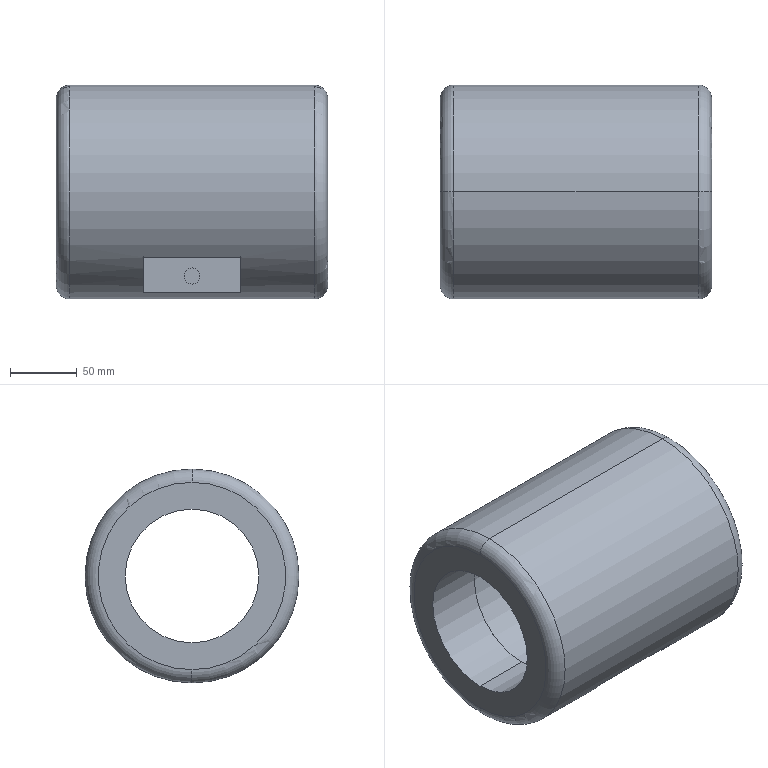Component | SolidWorks | CamMachineCasing-1 | 1 solid | 28 faces | box 203 x 160 x 160 mm | volume 2105138 mm3 | cylinder 10 | plane 10 | torus 8 | commonest cylinder face diameters 100 x4 12 x2 160 x2 112 x2
build123d program:
from build123d import *

# Parameters (mm, degrees)
SKETCH5_W          = 35
SKETCH5_H          = 72.809
CUT_EXTRUDE5_DEPTH = 120
SKETCH6_R          = 6
CUT_EXTRUDE6_DEPTH = 20


with BuildPart() as part:
    # Sketch1 → Revolve1 (revolve)
    with BuildSketch(Plane(origin=(0, 0, 0), x_dir=(0, 0, -1), z_dir=(1, 0, 0))):
        with BuildLine():
            Line((-56, -48), (-56, -155))
            ThreePointArc((-56, -155), (-54.828, -157.828), (-52, -159))
            Line((-52, -159), (-50, -159))
            Line((-50, -159), (-50, -203))
            Line((-50, -203), (-70, -203))
            ThreePointArc((-70, -203), (-77.071, -200.071), (-80, -193))
            Line((-80, -193), (-80, -10))
            ThreePointArc((-80, -10), (-77.071, -2.929), (-70, 0))
            Line((-70, 0), (-50, 0))
            Line((-50, 0), (-50, -44))
            Line((-50, -44), (-52, -44))
            ThreePointArc((-52, -44), (-54.828, -45.172), (-56, -48))
        make_face()
    revolve(axis=Axis((0, 0, 0), (0, -1, 0)))

    # Sketch5 → Cut-Extrude5 (cut)
    with BuildSketch(Plane(origin=(0, 0, -80), x_dir=(-1, 0, 0), z_dir=(0, 0, -1))):
        with Locations((45.79, -101.5)):
            Rectangle(SKETCH5_W, SKETCH5_H)
    extrude(amount=-CUT_EXTRUDE5_DEPTH, mode=Mode.SUBTRACT)

    # Sketch6 → Cut-Extrude6 (cut)
    with BuildSketch(Plane.ZY.offset(28.29)):
        with Locations((-62.831, -101.5)):
            Circle(SKETCH6_R)
    extrude(amount=-CUT_EXTRUDE6_DEPTH, mode=Mode.SUBTRACT)


solid = part.part

# Placed as in the assembly
solid = solid.moved(Location((587.733, 15.31, -110), (0, 0, 90)))
STEP:
#1=COLOUR_RGB('',0.7922,0.8196,0.9333);
#2=FILL_AREA_STYLE_COLOUR('',#1);
#3=FILL_AREA_STYLE('',(#2));
#4=SURFACE_STYLE_FILL_AREA(#3);
#5=SURFACE_SIDE_STYLE('',(#4));
#6=SURFACE_STYLE_USAGE(.BOTH.,#5);
#7=PRESENTATION_STYLE_ASSIGNMENT((#6));
#8=CARTESIAN_POINT('',(27.135,0.2764,-7.041));
#9=VERTEX_POINT('',#8);
#10=CARTESIAN_POINT('',(27.135,0.2764,-6.568));
#11=VERTEX_POINT('',#10);
#12=CARTESIAN_POINT('',(27.135,0.2764,-6.804));
#13=DIRECTION('',(0.,-1.,-0.));
#14=DIRECTION('',(0.,-0.,1.));
#15=AXIS2_PLACEMENT_3D('',#12,#13,#14);
#16=CIRCLE('',#15,0.2362);
#17=EDGE_CURVE('',#9,#11,#16,.T.);
#18=ORIENTED_EDGE('',*,*,#17,.F.);
#19=CARTESIAN_POINT('',(27.135,-0.511,-7.041));
#20=VERTEX_POINT('',#19);
#21=CARTESIAN_POINT('',(27.135,0.2764,-7.041));
#22=DIRECTION('',(0.,-1.,-0.));
#23=VECTOR('',#22,39.37);
#24=LINE('',#21,#23);
#25=EDGE_CURVE('',#9,#20,#24,.T.);
#26=ORIENTED_EDGE('',*,*,#25,.T.);
#27=CARTESIAN_POINT('',(27.135,-0.511,-6.568));
#28=VERTEX_POINT('',#27);
#29=CARTESIAN_POINT('',(27.135,-0.511,-6.804));
#30=DIRECTION('',(0.,-1.,-0.));
#31=DIRECTION('',(0.,0.,1.));
#32=AXIS2_PLACEMENT_3D('',#29,#30,#31);
#33=CIRCLE('',#32,0.2362);
#34=EDGE_CURVE('',#20,#28,#33,.T.);
#35=ORIENTED_EDGE('',*,*,#34,.T.);
#36=CARTESIAN_POINT('',(27.135,0.2764,-6.568));
#37=DIRECTION('',(0.,-1.,-0.));
#38=VECTOR('',#37,39.37);
#39=LINE('',#36,#38);
#40=EDGE_CURVE('',#11,#28,#39,.T.);
#41=ORIENTED_EDGE('',*,*,#40,.F.);
#42=EDGE_LOOP('',(#18,#26,#35,#41));
#43=FACE_OUTER_BOUND('',#42,.T.);
#44=CARTESIAN_POINT('',(27.135,0.2764,-6.804));
#45=DIRECTION('',(0.,-1.,-0.));
#46=DIRECTION('',(0.,-0.,1.));
#47=AXIS2_PLACEMENT_3D('',#44,#45,#46);
#48=CYLINDRICAL_SURFACE('',#47,0.2362);
#49=ADVANCED_FACE('',(#43),#48,.F.);
#50=CARTESIAN_POINT('',(29.399,0.6028,-6.378));
#51=VERTEX_POINT('',#50);
#52=CARTESIAN_POINT('',(29.399,0.6028,-2.283));
#53=VERTEX_POINT('',#52);
#54=CARTESIAN_POINT('',(29.399,0.6028,-4.331));
#55=DIRECTION('',(-1.,0.,0.));
#56=DIRECTION('',(0.,-0.,1.));
#57=AXIS2_PLACEMENT_3D('',#54,#55,#56);
#58=CIRCLE('',#57,2.047);
#59=EDGE_CURVE('',#51,#53,#58,.T.);
#60=ORIENTED_EDGE('',*,*,#59,.F.);
#61=CARTESIAN_POINT('',(29.241,0.6028,-6.535));
#62=VERTEX_POINT('',#61);
#63=CARTESIAN_POINT('',(29.241,0.6028,-6.378));
#64=DIRECTION('',(0.,1.,0.));
#65=DIRECTION('',(0.,-0.,1.));
#66=AXIS2_PLACEMENT_3D('',#63,#64,#65);
#67=CIRCLE('',#66,0.1575);
#68=EDGE_CURVE('',#51,#62,#67,.T.);
#69=ORIENTED_EDGE('',*,*,#68,.T.);
#70=CARTESIAN_POINT('',(29.241,0.6028,-2.126));
#71=VERTEX_POINT('',#70);
#72=CARTESIAN_POINT('',(29.241,0.6028,-4.331));
#73=DIRECTION('',(-1.,0.,0.));
#74=DIRECTION('',(0.,-0.,1.));
#75=AXIS2_PLACEMENT_3D('',#72,#73,#74);
#76=CIRCLE('',#75,2.205);
#77=EDGE_CURVE('',#62,#71,#76,.T.);
#78=ORIENTED_EDGE('',*,*,#77,.T.);
#79=CARTESIAN_POINT('',(29.241,0.6028,-2.283));
#80=DIRECTION('',(0.,-1.,-0.));
#81=DIRECTION('',(0.,0.,-1.));
#82=AXIS2_PLACEMENT_3D('',#79,#80,#81);
#83=CIRCLE('',#82,0.1575);
#84=EDGE_CURVE('',#53,#71,#83,.T.);
#85=ORIENTED_EDGE('',*,*,#84,.F.);
#86=EDGE_LOOP('',(#60,#69,#78,#85));
#87=FACE_OUTER_BOUND('',#86,.T.);
#88=CARTESIAN_POINT('',(29.241,0.6028,-4.331));
#89=DIRECTION('',(-1.,0.,0.));
#90=DIRECTION('',(0.,-0.,1.));
#91=AXIS2_PLACEMENT_3D('',#88,#89,#90);
#92=TOROIDAL_SURFACE('',#91,2.047,0.1575);
#93=ADVANCED_FACE('',(#87),#92,.F.);
#94=CARTESIAN_POINT('',(31.131,0.6028,-6.299));
#95=VERTEX_POINT('',#94);
#96=CARTESIAN_POINT('',(31.131,0.6028,-2.362));
#97=VERTEX_POINT('',#96);
#98=CARTESIAN_POINT('',(31.131,0.6028,-4.331));
#99=DIRECTION('',(-1.,0.,0.));
#100=DIRECTION('',(0.,-0.,1.));
#101=AXIS2_PLACEMENT_3D('',#98,#99,#100);
#102=CIRCLE('',#101,1.969);
#103=EDGE_CURVE('',#95,#97,#102,.T.);
#104=ORIENTED_EDGE('',*,*,#103,.F.);
#105=CARTESIAN_POINT('',(29.399,0.6028,-6.299));
#106=VERTEX_POINT('',#105);
#107=CARTESIAN_POINT('',(23.139,0.6028,-6.299));
#108=DIRECTION('',(-1.,0.,0.));
#109=VECTOR('',#108,39.37);
#110=LINE('',#107,#109);
#111=EDGE_CURVE('',#95,#106,#110,.T.);
#112=ORIENTED_EDGE('',*,*,#111,.T.);
#113=CARTESIAN_POINT('',(29.399,0.6028,-2.362));
#114=VERTEX_POINT('',#113);
#115=CARTESIAN_POINT('',(29.399,0.6028,-4.331));
#116=DIRECTION('',(-1.,0.,0.));
#117=DIRECTION('',(0.,-0.,1.));
#118=AXIS2_PLACEMENT_3D('',#115,#116,#117);
#119=CIRCLE('',#118,1.969);
#120=EDGE_CURVE('',#106,#114,#119,.T.);
#121=ORIENTED_EDGE('',*,*,#120,.T.);
#122=CARTESIAN_POINT('',(23.139,0.6028,-2.362));
#123=DIRECTION('',(-1.,0.,0.));
#124=VECTOR('',#123,39.37);
#125=LINE('',#122,#124);
#126=EDGE_CURVE('',#97,#114,#125,.T.);
#127=ORIENTED_EDGE('',*,*,#126,.F.);
#128=EDGE_LOOP('',(#104,#112,#121,#127));
#129=FACE_OUTER_BOUND('',#128,.T.);
#130=CARTESIAN_POINT('',(23.139,0.6028,-4.331));
#131=DIRECTION('',(-1.,0.,0.));
#132=DIRECTION('',(0.,-0.,1.));
#133=AXIS2_PLACEMENT_3D('',#130,#131,#132);
#134=CYLINDRICAL_SURFACE('',#133,1.969);
#135=ADVANCED_FACE('',(#129),#134,.F.);
#136=CARTESIAN_POINT('',(31.131,0.6028,-1.575));
#137=VERTEX_POINT('',#136);
#138=CARTESIAN_POINT('',(31.131,0.6028,-7.087));
#139=VERTEX_POINT('',#138);
#140=CARTESIAN_POINT('',(31.131,0.6028,-4.331));
#141=DIRECTION('',(-1.,0.,0.));
#142=DIRECTION('',(0.,-0.,1.));
#143=AXIS2_PLACEMENT_3D('',#140,#141,#142);
#144=CIRCLE('',#143,2.756);
#145=EDGE_CURVE('',#137,#139,#144,.T.);
#146=ORIENTED_EDGE('',*,*,#145,.T.);
#147=CARTESIAN_POINT('',(30.738,0.6028,-7.48));
#148=VERTEX_POINT('',#147);
#149=CARTESIAN_POINT('',(30.738,0.6028,-7.087));
#150=DIRECTION('',(0.,1.,0.));
#151=DIRECTION('',(0.,-0.,1.));
#152=AXIS2_PLACEMENT_3D('',#149,#150,#151);
#153=CIRCLE('',#152,0.3937);
#154=EDGE_CURVE('',#139,#148,#153,.T.);
#155=ORIENTED_EDGE('',*,*,#154,.T.);
#156=CARTESIAN_POINT('',(30.738,0.6028,-1.181));
#157=VERTEX_POINT('',#156);
#158=CARTESIAN_POINT('',(30.738,0.6028,-4.331));
#159=DIRECTION('',(-1.,0.,0.));
#160=DIRECTION('',(0.,-0.,1.));
#161=AXIS2_PLACEMENT_3D('',#158,#159,#160);
#162=CIRCLE('',#161,3.15);
#163=EDGE_CURVE('',#157,#148,#162,.T.);
#164=ORIENTED_EDGE('',*,*,#163,.F.);
#165=CARTESIAN_POINT('',(30.738,0.6028,-1.575));
#166=DIRECTION('',(0.,-1.,-0.));
#167=DIRECTION('',(0.,0.,-1.));
#168=AXIS2_PLACEMENT_3D('',#165,#166,#167);
#169=CIRCLE('',#168,0.3937);
#170=EDGE_CURVE('',#137,#157,#169,.T.);
#171=ORIENTED_EDGE('',*,*,#170,.F.);
#172=EDGE_LOOP('',(#146,#155,#164,#171));
#173=FACE_OUTER_BOUND('',#172,.T.);
#174=CARTESIAN_POINT('',(30.738,0.6028,-4.331));
#175=DIRECTION('',(-1.,0.,0.));
#176=DIRECTION('',(0.,-0.,1.));
#177=AXIS2_PLACEMENT_3D('',#174,#175,#176);
#178=TOROIDAL_SURFACE('',#177,2.756,0.3937);
#179=ADVANCED_FACE('',(#173),#178,.T.);
#180=ORIENTED_EDGE('',*,*,#163,.T.);
#181=CARTESIAN_POINT('',(23.533,0.6028,-7.48));
#182=VERTEX_POINT('',#181);
#183=CARTESIAN_POINT('',(23.139,0.6028,-7.48));
#184=DIRECTION('',(-1.,0.,0.));
#185=VECTOR('',#184,39.37);
#186=LINE('',#183,#185);
#187=EDGE_CURVE('',#148,#182,#186,.T.);
#188=ORIENTED_EDGE('',*,*,#187,.T.);
#189=CARTESIAN_POINT('',(23.533,0.6028,-1.181));
#190=VERTEX_POINT('',#189);
#191=CARTESIAN_POINT('',(23.533,0.6028,-4.331));
#192=DIRECTION('',(-1.,0.,0.));
#193=DIRECTION('',(0.,-0.,1.));
#194=AXIS2_PLACEMENT_3D('',#191,#192,#193);
#195=CIRCLE('',#194,3.15);
#196=EDGE_CURVE('',#190,#182,#195,.T.);
#197=ORIENTED_EDGE('',*,*,#196,.F.);
#198=CARTESIAN_POINT('',(23.139,0.6028,-1.181));
#199=DIRECTION('',(-1.,0.,0.));
#200=VECTOR('',#199,39.37);
#201=LINE('',#198,#200);
#202=EDGE_CURVE('',#157,#190,#201,.T.);
#203=ORIENTED_EDGE('',*,*,#202,.F.);
#204=EDGE_LOOP('',(#180,#188,#197,#203));
#205=FACE_OUTER_BOUND('',#204,.T.);
#206=CARTESIAN_POINT('',(23.139,0.6028,-4.331));
#207=DIRECTION('',(-1.,0.,0.));
#208=DIRECTION('',(0.,-0.,1.));
#209=AXIS2_PLACEMENT_3D('',#206,#207,#208);
#210=CYLINDRICAL_SURFACE('',#209,3.15);
#211=ADVANCED_FACE('',(#205),#210,.T.);
#212=ORIENTED_EDGE('',*,*,#196,.T.);
#213=CARTESIAN_POINT('',(23.139,0.6028,-7.087));
#214=VERTEX_POINT('',#213);
#215=CARTESIAN_POINT('',(23.533,0.6028,-7.087));
#216=DIRECTION('',(0.,1.,0.));
#217=DIRECTION('',(0.,-0.,1.));
#218=AXIS2_PLACEMENT_3D('',#215,#216,#217);
#219=CIRCLE('',#218,0.3937);
#220=EDGE_CURVE('',#182,#214,#219,.T.);
#221=ORIENTED_EDGE('',*,*,#220,.T.);
#222=CARTESIAN_POINT('',(23.139,0.6028,-1.575));
#223=VERTEX_POINT('',#222);
#224=CARTESIAN_POINT('',(23.139,0.6028,-4.331));
#225=DIRECTION('',(-1.,0.,0.));
#226=DIRECTION('',(0.,-0.,1.));
#227=AXIS2_PLACEMENT_3D('',#224,#225,#226);
#228=CIRCLE('',#227,2.756);
#229=EDGE_CURVE('',#223,#214,#228,.T.);
#230=ORIENTED_EDGE('',*,*,#229,.F.);
#231=CARTESIAN_POINT('',(23.533,0.6028,-1.575));
#232=DIRECTION('',(0.,-1.,-0.));
#233=DIRECTION('',(0.,0.,-1.));
#234=AXIS2_PLACEMENT_3D('',#231,#232,#233);
#235=CIRCLE('',#234,0.3937);
#236=EDGE_CURVE('',#190,#223,#235,.T.);
#237=ORIENTED_EDGE('',*,*,#236,.F.);
#238=EDGE_LOOP('',(#212,#221,#230,#237));
#239=FACE_OUTER_BOUND('',#238,.T.);
#240=CARTESIAN_POINT('',(23.533,0.6028,-4.331));
#241=DIRECTION('',(-1.,0.,0.));
#242=DIRECTION('',(0.,-0.,1.));
#243=AXIS2_PLACEMENT_3D('',#240,#241,#242);
#244=TOROIDAL_SURFACE('',#243,2.756,0.3937);
#245=ADVANCED_FACE('',(#239),#244,.T.);
#246=CARTESIAN_POINT('',(24.871,0.6028,-6.299));
#247=VERTEX_POINT('',#246);
#248=CARTESIAN_POINT('',(24.871,0.6028,-2.362));
#249=VERTEX_POINT('',#248);
#250=CARTESIAN_POINT('',(24.871,0.6028,-4.331));
#251=DIRECTION('',(-1.,0.,0.));
#252=DIRECTION('',(0.,-0.,1.));
#253=AXIS2_PLACEMENT_3D('',#250,#251,#252);
#254=CIRCLE('',#253,1.969);
#255=EDGE_CURVE('',#247,#249,#254,.T.);
#256=ORIENTED_EDGE('',*,*,#255,.F.);
#257=CARTESIAN_POINT('',(23.139,0.6028,-6.299));
#258=VERTEX_POINT('',#257);
#259=CARTESIAN_POINT('',(23.139,0.6028,-6.299));
#260=DIRECTION('',(-1.,0.,0.));
#261=VECTOR('',#260,39.37);
#262=LINE('',#259,#261);
#263=EDGE_CURVE('',#247,#258,#262,.T.);
#264=ORIENTED_EDGE('',*,*,#263,.T.);
#265=CARTESIAN_POINT('',(23.139,0.6028,-2.362));
#266=VERTEX_POINT('',#265);
#267=CARTESIAN_POINT('',(23.139,0.6028,-4.331));
#268=DIRECTION('',(-1.,0.,0.));
#269=DIRECTION('',(0.,-0.,1.));
#270=AXIS2_PLACEMENT_3D('',#267,#268,#269);
#271=CIRCLE('',#270,1.969);
#272=EDGE_CURVE('',#258,#266,#271,.T.);
#273=ORIENTED_EDGE('',*,*,#272,.T.);
#274=CARTESIAN_POINT('',(23.139,0.6028,-2.362));
#275=DIRECTION('',(-1.,0.,0.));
#276=VECTOR('',#275,39.37);
#277=LINE('',#274,#276);
#278=EDGE_CURVE('',#249,#266,#277,.T.);
#279=ORIENTED_EDGE('',*,*,#278,.F.);
#280=EDGE_LOOP('',(#256,#264,#273,#279));
#281=FACE_OUTER_BOUND('',#280,.T.);
#282=CARTESIAN_POINT('',(23.139,0.6028,-4.331));
#283=DIRECTION('',(-1.,0.,0.));
#284=DIRECTION('',(0.,-0.,1.));
#285=AXIS2_PLACEMENT_3D('',#282,#283,#284);
#286=CYLINDRICAL_SURFACE('',#285,1.969);
#287=ADVANCED_FACE('',(#281),#286,.F.);
#288=CARTESIAN_POINT('',(25.029,0.6028,-6.535));
#289=VERTEX_POINT('',#288);
#290=CARTESIAN_POINT('',(25.029,0.6028,-2.126));
#291=VERTEX_POINT('',#290);
#292=CARTESIAN_POINT('',(25.029,0.6028,-4.331));
#293=DIRECTION('',(-1.,0.,0.));
#294=DIRECTION('',(0.,-0.,1.));
#295=AXIS2_PLACEMENT_3D('',#292,#293,#294);
#296=CIRCLE('',#295,2.205);
#297=EDGE_CURVE('',#289,#291,#296,.T.);
#298=ORIENTED_EDGE('',*,*,#297,.F.);
#299=CARTESIAN_POINT('',(24.871,0.6028,-6.378));
#300=VERTEX_POINT('',#299);
#301=CARTESIAN_POINT('',(25.029,0.6028,-6.378));
#302=DIRECTION('',(0.,1.,0.));
#303=DIRECTION('',(0.,-0.,1.));
#304=AXIS2_PLACEMENT_3D('',#301,#302,#303);
#305=CIRCLE('',#304,0.1575);
#306=EDGE_CURVE('',#289,#300,#305,.T.);
#307=ORIENTED_EDGE('',*,*,#306,.T.);
#308=CARTESIAN_POINT('',(24.871,0.6028,-2.283));
#309=VERTEX_POINT('',#308);
#310=CARTESIAN_POINT('',(24.871,0.6028,-4.331));
#311=DIRECTION('',(-1.,0.,0.));
#312=DIRECTION('',(0.,-0.,1.));
#313=AXIS2_PLACEMENT_3D('',#310,#311,#312);
#314=CIRCLE('',#313,2.047);
#315=EDGE_CURVE('',#300,#309,#314,.T.);
#316=ORIENTED_EDGE('',*,*,#315,.T.);
#317=CARTESIAN_POINT('',(25.029,0.6028,-2.283));
#318=DIRECTION('',(0.,-1.,-0.));
#319=DIRECTION('',(0.,0.,-1.));
#320=AXIS2_PLACEMENT_3D('',#317,#318,#319);
#321=CIRCLE('',#320,0.1575);
#322=EDGE_CURVE('',#291,#309,#321,.T.);
#323=ORIENTED_EDGE('',*,*,#322,.F.);
#324=EDGE_LOOP('',(#298,#307,#316,#323));
#325=FACE_OUTER_BOUND('',#324,.T.);
#326=CARTESIAN_POINT('',(25.029,0.6028,-4.331));
#327=DIRECTION('',(-1.,0.,0.));
#328=DIRECTION('',(0.,-0.,1.));
#329=AXIS2_PLACEMENT_3D('',#326,#327,#328);
#330=TOROIDAL_SURFACE('',#329,2.047,0.1575);
#331=ADVANCED_FACE('',(#325),#330,.F.);
#332=CARTESIAN_POINT('',(25.702,-0.9402,-2.756));
#333=VERTEX_POINT('',#332);
#334=CARTESIAN_POINT('',(25.702,-0.511,-6.233));
#335=VERTEX_POINT('',#334);
#336=CARTESIAN_POINT('',(25.702,0.6028,-4.331));
#337=DIRECTION('',(1.,-0.,-0.));
#338=DIRECTION('',(0.,-1.,-0.));
#339=AXIS2_PLACEMENT_3D('',#336,#337,#338);
#340=CIRCLE('',#339,2.205);
#341=EDGE_CURVE('',#333,#335,#340,.T.);
#342=ORIENTED_EDGE('',*,*,#341,.T.);
#343=CARTESIAN_POINT('',(28.568,-0.511,-6.233));
#344=VERTEX_POINT('',#343);
#345=CARTESIAN_POINT('',(23.139,-0.511,-6.233));
#346=DIRECTION('',(1.,0.,0.));
#347=VECTOR('',#346,39.37);
#348=LINE('',#345,#347);
#349=EDGE_CURVE('',#335,#344,#348,.T.);
#350=ORIENTED_EDGE('',*,*,#349,.T.);
#351=CARTESIAN_POINT('',(28.568,-0.9402,-2.756));
#352=VERTEX_POINT('',#351);
#353=CARTESIAN_POINT('',(28.568,0.6028,-4.331));
#354=DIRECTION('',(-1.,0.,0.));
#355=DIRECTION('',(0.,0.,-1.));
#356=AXIS2_PLACEMENT_3D('',#353,#354,#355);
#357=CIRCLE('',#356,2.205);
#358=EDGE_CURVE('',#344,#352,#357,.T.);
#359=ORIENTED_EDGE('',*,*,#358,.T.);
#360=CARTESIAN_POINT('',(23.139,-0.9402,-2.756));
#361=DIRECTION('',(-1.,0.,0.));
#362=VECTOR('',#361,39.37);
#363=LINE('',#360,#362);
#364=EDGE_CURVE('',#352,#333,#363,.T.);
#365=ORIENTED_EDGE('',*,*,#364,.T.);
#366=EDGE_LOOP('',(#342,#350,#359,#365));
#367=FACE_BOUND('',#366,.T.);
#368=ORIENTED_EDGE('',*,*,#77,.F.);
#369=CARTESIAN_POINT('',(23.139,0.6028,-6.535));
#370=DIRECTION('',(-1.,0.,0.));
#371=VECTOR('',#370,39.37);
#372=LINE('',#369,#371);
#373=EDGE_CURVE('',#62,#289,#372,.T.);
#374=ORIENTED_EDGE('',*,*,#373,.T.);
#375=ORIENTED_EDGE('',*,*,#297,.T.);
#376=CARTESIAN_POINT('',(23.139,0.6028,-2.126));
#377=DIRECTION('',(-1.,0.,0.));
#378=VECTOR('',#377,39.37);
#379=LINE('',#376,#378);
#380=EDGE_CURVE('',#71,#291,#379,.T.);
#381=ORIENTED_EDGE('',*,*,#380,.F.);
#382=EDGE_LOOP('',(#368,#374,#375,#381));
#383=FACE_OUTER_BOUND('',#382,.T.);
#384=CARTESIAN_POINT('',(23.139,0.6028,-4.331));
#385=DIRECTION('',(-1.,0.,0.));
#386=DIRECTION('',(0.,-0.,1.));
#387=AXIS2_PLACEMENT_3D('',#384,#385,#386);
#388=CYLINDRICAL_SURFACE('',#387,2.205);
#389=ADVANCED_FACE('',(#367,#383),#388,.F.);
#390=ORIENTED_EDGE('',*,*,#373,.F.);
#391=CARTESIAN_POINT('',(29.241,0.6028,-4.331));
#392=DIRECTION('',(-1.,0.,0.));
#393=DIRECTION('',(0.,-0.,1.));
#394=AXIS2_PLACEMENT_3D('',#391,#392,#393);
#395=CIRCLE('',#394,2.205);
#396=EDGE_CURVE('',#71,#62,#395,.T.);
#397=ORIENTED_EDGE('',*,*,#396,.F.);
#398=ORIENTED_EDGE('',*,*,#380,.T.);
#399=CARTESIAN_POINT('',(25.029,0.6028,-4.331));
#400=DIRECTION('',(-1.,0.,0.));
#401=DIRECTION('',(0.,-0.,1.));
#402=AXIS2_PLACEMENT_3D('',#399,#400,#401);
#403=CIRCLE('',#402,2.205);
#404=EDGE_CURVE('',#291,#289,#403,.T.);
#405=ORIENTED_EDGE('',*,*,#404,.T.);
#406=EDGE_LOOP('',(#390,#397,#398,#405));
#407=FACE_OUTER_BOUND('',#406,.T.);
#408=CARTESIAN_POINT('',(23.139,0.6028,-4.331));
#409=DIRECTION('',(-1.,0.,0.));
#410=DIRECTION('',(0.,-0.,1.));
#411=AXIS2_PLACEMENT_3D('',#408,#409,#410);
#412=CYLINDRICAL_SURFACE('',#411,2.205);
#413=ADVANCED_FACE('',(#407),#412,.F.);
#414=ORIENTED_EDGE('',*,*,#306,.F.);
#415=ORIENTED_EDGE('',*,*,#404,.F.);
#416=ORIENTED_EDGE('',*,*,#322,.T.);
#417=CARTESIAN_POINT('',(24.871,0.6028,-4.331));
#418=DIRECTION('',(-1.,0.,0.));
#419=DIRECTION('',(0.,-0.,1.));
#420=AXIS2_PLACEMENT_3D('',#417,#418,#419);
#421=CIRCLE('',#420,2.047);
#422=EDGE_CURVE('',#309,#300,#421,.T.);
#423=ORIENTED_EDGE('',*,*,#422,.T.);
#424=EDGE_LOOP('',(#414,#415,#416,#423));
#425=FACE_OUTER_BOUND('',#424,.T.);
#426=CARTESIAN_POINT('',(25.029,0.6028,-4.331));
#427=DIRECTION('',(-1.,0.,0.));
#428=DIRECTION('',(0.,-0.,1.));
#429=AXIS2_PLACEMENT_3D('',#426,#427,#428);
#430=TOROIDAL_SURFACE('',#429,2.047,0.1575);
#431=ADVANCED_FACE('',(#425),#430,.F.);
#432=ORIENTED_EDGE('',*,*,#422,.F.);
#433=ORIENTED_EDGE('',*,*,#315,.F.);
#434=EDGE_LOOP('',(#432,#433));
#435=FACE_OUTER_BOUND('',#434,.T.);
#436=CARTESIAN_POINT('',(24.871,0.6028,-4.331));
#437=DIRECTION('',(-1.,0.,0.));
#438=DIRECTION('',(0.,-0.,1.));
#439=AXIS2_PLACEMENT_3D('',#436,#437,#438);
#440=CIRCLE('',#439,1.969);
#441=EDGE_CURVE('',#249,#247,#440,.T.);
#442=ORIENTED_EDGE('',*,*,#441,.T.);
#443=ORIENTED_EDGE('',*,*,#255,.T.);
#444=EDGE_LOOP('',(#442,#443));
#445=FACE_BOUND('',#444,.T.);
#446=CARTESIAN_POINT('',(24.871,0.6028,-4.331));
#447=DIRECTION('',(-1.,0.,0.));
#448=DIRECTION('',(0.,-0.,1.));
#449=AXIS2_PLACEMENT_3D('',#446,#447,#448);
#450=PLANE('',#449);
#451=ADVANCED_FACE('',(#435,#445),#450,.F.);
#452=ORIENTED_EDGE('',*,*,#263,.F.);
#453=ORIENTED_EDGE('',*,*,#441,.F.);
#454=ORIENTED_EDGE('',*,*,#278,.T.);
#455=CARTESIAN_POINT('',(23.139,0.6028,-4.331));
#456=DIRECTION('',(-1.,0.,0.));
#457=DIRECTION('',(0.,-0.,1.));
#458=AXIS2_PLACEMENT_3D('',#455,#456,#457);
#459=CIRCLE('',#458,1.969);
#460=EDGE_CURVE('',#266,#258,#459,.T.);
#461=ORIENTED_EDGE('',*,*,#460,.T.);
#462=EDGE_LOOP('',(#452,#453,#454,#461));
#463=FACE_OUTER_BOUND('',#462,.T.);
#464=CARTESIAN_POINT('',(23.139,0.6028,-4.331));
#465=DIRECTION('',(-1.,0.,0.));
#466=DIRECTION('',(0.,-0.,1.));
#467=AXIS2_PLACEMENT_3D('',#464,#465,#466);
#468=CYLINDRICAL_SURFACE('',#467,1.969);
#469=ADVANCED_FACE('',(#463),#468,.F.);
#470=ORIENTED_EDGE('',*,*,#229,.T.);
#471=CARTESIAN_POINT('',(23.139,0.6028,-4.331));
#472=DIRECTION('',(-1.,0.,0.));
#473=DIRECTION('',(0.,-0.,1.));
#474=AXIS2_PLACEMENT_3D('',#471,#472,#473);
#475=CIRCLE('',#474,2.756);
#476=EDGE_CURVE('',#214,#223,#475,.T.);
#477=ORIENTED_EDGE('',*,*,#476,.T.);
#478=EDGE_LOOP('',(#470,#477));
#479=FACE_OUTER_BOUND('',#478,.T.);
#480=ORIENTED_EDGE('',*,*,#460,.F.);
#481=ORIENTED_EDGE('',*,*,#272,.F.);
#482=EDGE_LOOP('',(#480,#481));
#483=FACE_BOUND('',#482,.T.);
#484=CARTESIAN_POINT('',(23.139,0.6028,-4.331));
#485=DIRECTION('',(-1.,0.,0.));
#486=DIRECTION('',(0.,-0.,1.));
#487=AXIS2_PLACEMENT_3D('',#484,#485,#486);
#488=PLANE('',#487);
#489=ADVANCED_FACE('',(#479,#483),#488,.T.);
#490=ORIENTED_EDGE('',*,*,#220,.F.);
#491=CARTESIAN_POINT('',(23.533,0.6028,-4.331));
#492=DIRECTION('',(-1.,0.,0.));
#493=DIRECTION('',(0.,-0.,1.));
#494=AXIS2_PLACEMENT_3D('',#491,#492,#493);
#495=CIRCLE('',#494,3.15);
#496=EDGE_CURVE('',#182,#190,#495,.T.);
#497=ORIENTED_EDGE('',*,*,#496,.T.);
#498=ORIENTED_EDGE('',*,*,#236,.T.);
#499=ORIENTED_EDGE('',*,*,#476,.F.);
#500=EDGE_LOOP('',(#490,#497,#498,#499));
#501=FACE_OUTER_BOUND('',#500,.T.);
#502=CARTESIAN_POINT('',(23.533,0.6028,-4.331));
#503=DIRECTION('',(-1.,0.,0.));
#504=DIRECTION('',(0.,-0.,1.));
#505=AXIS2_PLACEMENT_3D('',#502,#503,#504);
#506=TOROIDAL_SURFACE('',#505,2.756,0.3937);
#507=ADVANCED_FACE('',(#501),#506,.T.);
#508=ORIENTED_EDGE('',*,*,#187,.F.);
#509=CARTESIAN_POINT('',(30.738,0.6028,-4.331));
#510=DIRECTION('',(-1.,0.,0.));
#511=DIRECTION('',(0.,-0.,1.));
#512=AXIS2_PLACEMENT_3D('',#509,#510,#511);
#513=CIRCLE('',#512,3.15);
#514=EDGE_CURVE('',#148,#157,#513,.T.);
#515=ORIENTED_EDGE('',*,*,#514,.T.);
#516=ORIENTED_EDGE('',*,*,#202,.T.);
#517=ORIENTED_EDGE('',*,*,#496,.F.);
#518=EDGE_LOOP('',(#508,#515,#516,#517));
#519=FACE_OUTER_BOUND('',#518,.T.);
#520=CARTESIAN_POINT('',(25.702,-0.511,-7.277));
#521=VERTEX_POINT('',#520);
#522=CARTESIAN_POINT('',(28.568,-0.511,-7.277));
#523=VERTEX_POINT('',#522);
#524=CARTESIAN_POINT('',(23.139,-0.511,-7.277));
#525=DIRECTION('',(1.,0.,0.));
#526=VECTOR('',#525,39.37);
#527=LINE('',#524,#526);
#528=EDGE_CURVE('',#521,#523,#527,.T.);
#529=ORIENTED_EDGE('',*,*,#528,.F.);
#530=CARTESIAN_POINT('',(25.702,-1.889,-6.257));
#531=VERTEX_POINT('',#530);
#532=CARTESIAN_POINT('',(25.702,0.6028,-4.331));
#533=DIRECTION('',(1.,-0.,-0.));
#534=DIRECTION('',(0.,-1.,0.));
#535=AXIS2_PLACEMENT_3D('',#532,#533,#534);
#536=CIRCLE('',#535,3.15);
#537=EDGE_CURVE('',#531,#521,#536,.T.);
#538=ORIENTED_EDGE('',*,*,#537,.F.);
#539=CARTESIAN_POINT('',(28.568,-1.889,-6.257));
#540=VERTEX_POINT('',#539);
#541=CARTESIAN_POINT('',(23.139,-1.889,-6.257));
#542=DIRECTION('',(-1.,0.,0.));
#543=VECTOR('',#542,39.37);
#544=LINE('',#541,#543);
#545=EDGE_CURVE('',#540,#531,#544,.T.);
#546=ORIENTED_EDGE('',*,*,#545,.F.);
#547=CARTESIAN_POINT('',(28.568,0.6028,-4.331));
#548=DIRECTION('',(-1.,0.,0.));
#549=DIRECTION('',(0.,0.,-1.));
#550=AXIS2_PLACEMENT_3D('',#547,#548,#549);
#551=CIRCLE('',#550,3.15);
#552=EDGE_CURVE('',#523,#540,#551,.T.);
#553=ORIENTED_EDGE('',*,*,#552,.F.);
#554=EDGE_LOOP('',(#529,#538,#546,#553));
#555=FACE_BOUND('',#554,.T.);
#556=CARTESIAN_POINT('',(23.139,0.6028,-4.331));
#557=DIRECTION('',(-1.,0.,0.));
#558=DIRECTION('',(0.,-0.,1.));
#559=AXIS2_PLACEMENT_3D('',#556,#557,#558);
#560=CYLINDRICAL_SURFACE('',#559,3.15);
#561=ADVANCED_FACE('',(#519,#555),#560,.T.);
#562=ORIENTED_EDGE('',*,*,#154,.F.);
#563=CARTESIAN_POINT('',(31.131,0.6028,-4.331));
#564=DIRECTION('',(-1.,0.,0.));
#565=DIRECTION('',(0.,-0.,1.));
#566=AXIS2_PLACEMENT_3D('',#563,#564,#565);
#567=CIRCLE('',#566,2.756);
#568=EDGE_CURVE('',#139,#137,#567,.T.);
#569=ORIENTED_EDGE('',*,*,#568,.T.);
#570=ORIENTED_EDGE('',*,*,#170,.T.);
#571=ORIENTED_EDGE('',*,*,#514,.F.);
#572=EDGE_LOOP('',(#562,#569,#570,#571));
#573=FACE_OUTER_BOUND('',#572,.T.);
#574=CARTESIAN_POINT('',(30.738,0.6028,-4.331));
#575=DIRECTION('',(-1.,0.,0.));
#576=DIRECTION('',(0.,-0.,1.));
#577=AXIS2_PLACEMENT_3D('',#574,#575,#576);
#578=TOROIDAL_SURFACE('',#577,2.756,0.3937);
#579=ADVANCED_FACE('',(#573),#578,.T.);
#580=CARTESIAN_POINT('',(31.131,0.6028,-4.331));
#581=DIRECTION('',(-1.,0.,0.));
#582=DIRECTION('',(0.,-0.,1.));
#583=AXIS2_PLACEMENT_3D('',#580,#581,#582);
#584=CIRCLE('',#583,1.969);
#585=EDGE_CURVE('',#97,#95,#584,.T.);
#586=ORIENTED_EDGE('',*,*,#585,.T.);
#587=ORIENTED_EDGE('',*,*,#103,.T.);
#588=EDGE_LOOP('',(#586,#587));
#589=FACE_BOUND('',#588,.T.);
#590=ORIENTED_EDGE('',*,*,#145,.F.);
#591=ORIENTED_EDGE('',*,*,#568,.F.);
#592=EDGE_LOOP('',(#590,#591));
#593=FACE_OUTER_BOUND('',#592,.T.);
#594=CARTESIAN_POINT('',(31.131,0.6028,-4.331));
#595=DIRECTION('',(1.,0.,0.));
#596=DIRECTION('',(0.,0.,-1.));
#597=AXIS2_PLACEMENT_3D('',#594,#595,#596);
#598=PLANE('',#597);
#599=ADVANCED_FACE('',(#589,#593),#598,.T.);
#600=ORIENTED_EDGE('',*,*,#111,.F.);
#601=ORIENTED_EDGE('',*,*,#585,.F.);
#602=ORIENTED_EDGE('',*,*,#126,.T.);
#603=CARTESIAN_POINT('',(29.399,0.6028,-4.331));
#604=DIRECTION('',(-1.,0.,0.));
#605=DIRECTION('',(0.,-0.,1.));
#606=AXIS2_PLACEMENT_3D('',#603,#604,#605);
#607=CIRCLE('',#606,1.969);
#608=EDGE_CURVE('',#114,#106,#607,.T.);
#609=ORIENTED_EDGE('',*,*,#608,.T.);
#610=EDGE_LOOP('',(#600,#601,#602,#609));
#611=FACE_OUTER_BOUND('',#610,.T.);
#612=CARTESIAN_POINT('',(23.139,0.6028,-4.331));
#613=DIRECTION('',(-1.,0.,0.));
#614=DIRECTION('',(0.,-0.,1.));
#615=AXIS2_PLACEMENT_3D('',#612,#613,#614);
#616=CYLINDRICAL_SURFACE('',#615,1.969);
#617=ADVANCED_FACE('',(#611),#616,.F.);
#618=ORIENTED_EDGE('',*,*,#608,.F.);
#619=ORIENTED_EDGE('',*,*,#120,.F.);
#620=EDGE_LOOP('',(#618,#619));
#621=FACE_BOUND('',#620,.T.);
#622=CARTESIAN_POINT('',(29.399,0.6028,-4.331));
#623=DIRECTION('',(-1.,0.,0.));
#624=DIRECTION('',(0.,-0.,1.));
#625=AXIS2_PLACEMENT_3D('',#622,#623,#624);
#626=CIRCLE('',#625,2.047);
#627=EDGE_CURVE('',#53,#51,#626,.T.);
#628=ORIENTED_EDGE('',*,*,#627,.T.);
#629=ORIENTED_EDGE('',*,*,#59,.T.);
#630=EDGE_LOOP('',(#628,#629));
#631=FACE_OUTER_BOUND('',#630,.T.);
#632=CARTESIAN_POINT('',(29.399,0.6028,-4.331));
#633=DIRECTION('',(1.,0.,0.));
#634=DIRECTION('',(0.,0.,-1.));
#635=AXIS2_PLACEMENT_3D('',#632,#633,#634);
#636=PLANE('',#635);
#637=ADVANCED_FACE('',(#621,#631),#636,.F.);
#638=ORIENTED_EDGE('',*,*,#68,.F.);
#639=ORIENTED_EDGE('',*,*,#627,.F.);
#640=ORIENTED_EDGE('',*,*,#84,.T.);
#641=ORIENTED_EDGE('',*,*,#396,.T.);
#642=EDGE_LOOP('',(#638,#639,#640,#641));
#643=FACE_OUTER_BOUND('',#642,.T.);
#644=CARTESIAN_POINT('',(29.241,0.6028,-4.331));
#645=DIRECTION('',(-1.,0.,0.));
#646=DIRECTION('',(0.,-0.,1.));
#647=AXIS2_PLACEMENT_3D('',#644,#645,#646);
#648=TOROIDAL_SURFACE('',#647,2.047,0.1575);
#649=ADVANCED_FACE('',(#643),#648,.F.);
#650=CARTESIAN_POINT('',(28.568,-1.889,-2.756));
#651=VERTEX_POINT('',#650);
#652=CARTESIAN_POINT('',(28.568,-1.889,-2.756));
#653=DIRECTION('',(0.,-1.,-0.));
#654=VECTOR('',#653,39.37);
#655=LINE('',#652,#654);
#656=EDGE_CURVE('',#352,#651,#655,.T.);
#657=ORIENTED_EDGE('',*,*,#656,.T.);
#658=CARTESIAN_POINT('',(25.702,-1.889,-2.756));
#659=VERTEX_POINT('',#658);
#660=CARTESIAN_POINT('',(25.702,-1.889,-2.756));
#661=DIRECTION('',(-1.,0.,0.));
#662=VECTOR('',#661,39.37);
#663=LINE('',#660,#662);
#664=EDGE_CURVE('',#651,#659,#663,.T.);
#665=ORIENTED_EDGE('',*,*,#664,.T.);
#666=CARTESIAN_POINT('',(25.702,-1.889,-2.756));
#667=DIRECTION('',(0.,1.,0.));
#668=VECTOR('',#667,39.37);
#669=LINE('',#666,#668);
#670=EDGE_CURVE('',#659,#333,#669,.T.);
#671=ORIENTED_EDGE('',*,*,#670,.T.);
#672=ORIENTED_EDGE('',*,*,#364,.F.);
#673=EDGE_LOOP('',(#657,#665,#671,#672));
#674=FACE_OUTER_BOUND('',#673,.T.);
#675=CARTESIAN_POINT('',(23.139,0.6028,-2.756));
#676=DIRECTION('',(0.,-0.,1.));
#677=DIRECTION('',(0.,1.,0.));
#678=AXIS2_PLACEMENT_3D('',#675,#676,#677);
#679=PLANE('',#678);
#680=ADVANCED_FACE('',(#674),#679,.F.);
#681=CARTESIAN_POINT('',(27.135,-0.511,-6.804));
#682=DIRECTION('',(0.,-1.,-0.));
#683=DIRECTION('',(0.,0.,1.));
#684=AXIS2_PLACEMENT_3D('',#681,#682,#683);
#685=CIRCLE('',#684,0.2362);
#686=EDGE_CURVE('',#28,#20,#685,.T.);
#687=ORIENTED_EDGE('',*,*,#686,.F.);
#688=ORIENTED_EDGE('',*,*,#34,.F.);
#689=EDGE_LOOP('',(#687,#688));
#690=FACE_BOUND('',#689,.T.);
#691=CARTESIAN_POINT('',(25.702,-0.511,-2.756));
#692=DIRECTION('',(0.,0.,-1.));
#693=VECTOR('',#692,39.37);
#694=LINE('',#691,#693);
#695=EDGE_CURVE('',#335,#521,#694,.T.);
#696=ORIENTED_EDGE('',*,*,#695,.T.);
#697=ORIENTED_EDGE('',*,*,#528,.T.);
#698=CARTESIAN_POINT('',(28.568,-0.511,-2.756));
#699=DIRECTION('',(0.,0.,-1.));
#700=VECTOR('',#699,39.37);
#701=LINE('',#698,#700);
#702=EDGE_CURVE('',#344,#523,#701,.T.);
#703=ORIENTED_EDGE('',*,*,#702,.F.);
#704=ORIENTED_EDGE('',*,*,#349,.F.);
#705=EDGE_LOOP('',(#696,#697,#703,#704));
#706=FACE_OUTER_BOUND('',#705,.T.);
#707=CARTESIAN_POINT('',(25.702,-0.511,-2.756));
#708=DIRECTION('',(0.,1.,0.));
#709=DIRECTION('',(0.,0.,-1.));
#710=AXIS2_PLACEMENT_3D('',#707,#708,#709);
#711=PLANE('',#710);
#712=ADVANCED_FACE('',(#690,#706),#711,.F.);
#713=ORIENTED_EDGE('',*,*,#670,.F.);
#714=CARTESIAN_POINT('',(25.702,-1.889,-2.756));
#715=DIRECTION('',(0.,0.,-1.));
#716=VECTOR('',#715,39.37);
#717=LINE('',#714,#716);
#718=EDGE_CURVE('',#659,#531,#717,.T.);
#719=ORIENTED_EDGE('',*,*,#718,.T.);
#720=ORIENTED_EDGE('',*,*,#537,.T.);
#721=ORIENTED_EDGE('',*,*,#695,.F.);
#722=ORIENTED_EDGE('',*,*,#341,.F.);
#723=EDGE_LOOP('',(#713,#719,#720,#721,#722));
#724=FACE_OUTER_BOUND('',#723,.T.);
#725=CARTESIAN_POINT('',(25.702,-1.889,-2.756));
#726=DIRECTION('',(-1.,0.,0.));
#727=DIRECTION('',(-0.,-1.,-0.));
#728=AXIS2_PLACEMENT_3D('',#725,#726,#727);
#729=PLANE('',#728);
#730=ADVANCED_FACE('',(#724),#729,.F.);
#731=ORIENTED_EDGE('',*,*,#702,.T.);
#732=ORIENTED_EDGE('',*,*,#552,.T.);
#733=CARTESIAN_POINT('',(28.568,-1.889,-2.756));
#734=DIRECTION('',(0.,0.,-1.));
#735=VECTOR('',#734,39.37);
#736=LINE('',#733,#735);
#737=EDGE_CURVE('',#651,#540,#736,.T.);
#738=ORIENTED_EDGE('',*,*,#737,.F.);
#739=ORIENTED_EDGE('',*,*,#656,.F.);
#740=ORIENTED_EDGE('',*,*,#358,.F.);
#741=EDGE_LOOP('',(#731,#732,#738,#739,#740));
#742=FACE_OUTER_BOUND('',#741,.T.);
#743=CARTESIAN_POINT('',(28.568,-1.889,-2.756));
#744=DIRECTION('',(1.,0.,0.));
#745=DIRECTION('',(0.,0.,-1.));
#746=AXIS2_PLACEMENT_3D('',#743,#744,#745);
#747=PLANE('',#746);
#748=ADVANCED_FACE('',(#742),#747,.F.);
#749=ORIENTED_EDGE('',*,*,#545,.T.);
#750=ORIENTED_EDGE('',*,*,#718,.F.);
#751=ORIENTED_EDGE('',*,*,#664,.F.);
#752=ORIENTED_EDGE('',*,*,#737,.T.);
#753=EDGE_LOOP('',(#749,#750,#751,#752));
#754=FACE_OUTER_BOUND('',#753,.T.);
#755=CARTESIAN_POINT('',(25.702,-1.889,-2.756));
#756=DIRECTION('',(-0.,-1.,-0.));
#757=DIRECTION('',(1.,-0.,-0.));
#758=AXIS2_PLACEMENT_3D('',#755,#756,#757);
#759=PLANE('',#758);
#760=ADVANCED_FACE('',(#754),#759,.F.);
#761=ORIENTED_EDGE('',*,*,#25,.F.);
#762=CARTESIAN_POINT('',(27.135,0.2764,-6.804));
#763=DIRECTION('',(0.,-1.,-0.));
#764=DIRECTION('',(0.,-0.,1.));
#765=AXIS2_PLACEMENT_3D('',#762,#763,#764);
#766=CIRCLE('',#765,0.2362);
#767=EDGE_CURVE('',#11,#9,#766,.T.);
#768=ORIENTED_EDGE('',*,*,#767,.F.);
#769=ORIENTED_EDGE('',*,*,#40,.T.);
#770=ORIENTED_EDGE('',*,*,#686,.T.);
#771=EDGE_LOOP('',(#761,#768,#769,#770));
#772=FACE_OUTER_BOUND('',#771,.T.);
#773=CARTESIAN_POINT('',(27.135,0.2764,-6.804));
#774=DIRECTION('',(0.,-1.,-0.));
#775=DIRECTION('',(0.,-0.,1.));
#776=AXIS2_PLACEMENT_3D('',#773,#774,#775);
#777=CYLINDRICAL_SURFACE('',#776,0.2362);
#778=ADVANCED_FACE('',(#772),#777,.F.);
#779=ORIENTED_EDGE('',*,*,#767,.T.);
#780=ORIENTED_EDGE('',*,*,#17,.T.);
#781=EDGE_LOOP('',(#779,#780));
#782=FACE_OUTER_BOUND('',#781,.T.);
#783=CARTESIAN_POINT('',(27.135,0.2764,-6.804));
#784=DIRECTION('',(0.,-1.,-0.));
#785=DIRECTION('',(0.,-0.,1.));
#786=AXIS2_PLACEMENT_3D('',#783,#784,#785);
#787=PLANE('',#786);
#788=ADVANCED_FACE('',(#782),#787,.T.);
#789=CLOSED_SHELL('',(#49,#93,#135,#179,#211,#245,#287,#331,#389,#413,#431,#451,#469,#489,#507,#561,#579,#599,#617,#637,#649,#680,#712,#730,#748,#760,#778,#788));
#790=MANIFOLD_SOLID_BREP('',#789);
#791=STYLED_ITEM('',(#7),#790);
#792=(LENGTH_UNIT()NAMED_UNIT(*)SI_UNIT($,.METRE.));
#793=LENGTH_MEASURE_WITH_UNIT(LENGTH_MEASURE(0.0254),#792);
#794=DIMENSIONAL_EXPONENTS(1.,0.,0.,0.,0.,0.,0.);
#795=(CONVERSION_BASED_UNIT('',#793)LENGTH_UNIT()NAMED_UNIT(#794));
#796=UNCERTAINTY_MEASURE_WITH_UNIT(LENGTH_MEASURE(0.00001),#795,'','');
#797=(NAMED_UNIT(*)PLANE_ANGLE_UNIT()SI_UNIT($,.RADIAN.));
#798=(NAMED_UNIT(*)SI_UNIT($,.STERADIAN.)SOLID_ANGLE_UNIT());
#799=(GEOMETRIC_REPRESENTATION_CONTEXT(3)GLOBAL_UNCERTAINTY_ASSIGNED_CONTEXT((#796))GLOBAL_UNIT_ASSIGNED_CONTEXT((#795,#797,#798))REPRESENTATION_CONTEXT('',''));
#800=MECHANICAL_DESIGN_GEOMETRIC_PRESENTATION_REPRESENTATION('',(#791),#799);
#801=PRESENTATION_LAYER_ASSIGNMENT('','',(#791));
#802=CARTESIAN_POINT('',(0.,0.,0.));
#803=DIRECTION('',(0.,0.,1.));
#804=DIRECTION('',(1.,0.,0.));
#805=AXIS2_PLACEMENT_3D('',#802,#803,#804);
#806=(LENGTH_UNIT()NAMED_UNIT(*)SI_UNIT($,.METRE.));
#807=LENGTH_MEASURE_WITH_UNIT(LENGTH_MEASURE(0.0254),#806);
#808=DIMENSIONAL_EXPONENTS(1.,0.,0.,0.,0.,0.,0.);
#809=(CONVERSION_BASED_UNIT('',#807)LENGTH_UNIT()NAMED_UNIT(#808));
#810=UNCERTAINTY_MEASURE_WITH_UNIT(LENGTH_MEASURE(0.00001),#809,'','');
#811=(NAMED_UNIT(*)PLANE_ANGLE_UNIT()SI_UNIT($,.RADIAN.));
#812=(NAMED_UNIT(*)SI_UNIT($,.STERADIAN.)SOLID_ANGLE_UNIT());
#813=(GEOMETRIC_REPRESENTATION_CONTEXT(3)GLOBAL_UNCERTAINTY_ASSIGNED_CONTEXT((#810))GLOBAL_UNIT_ASSIGNED_CONTEXT((#809,#811,#812))REPRESENTATION_CONTEXT('',''));
#814=ADVANCED_BREP_SHAPE_REPRESENTATION('',(#790,#805),#813);